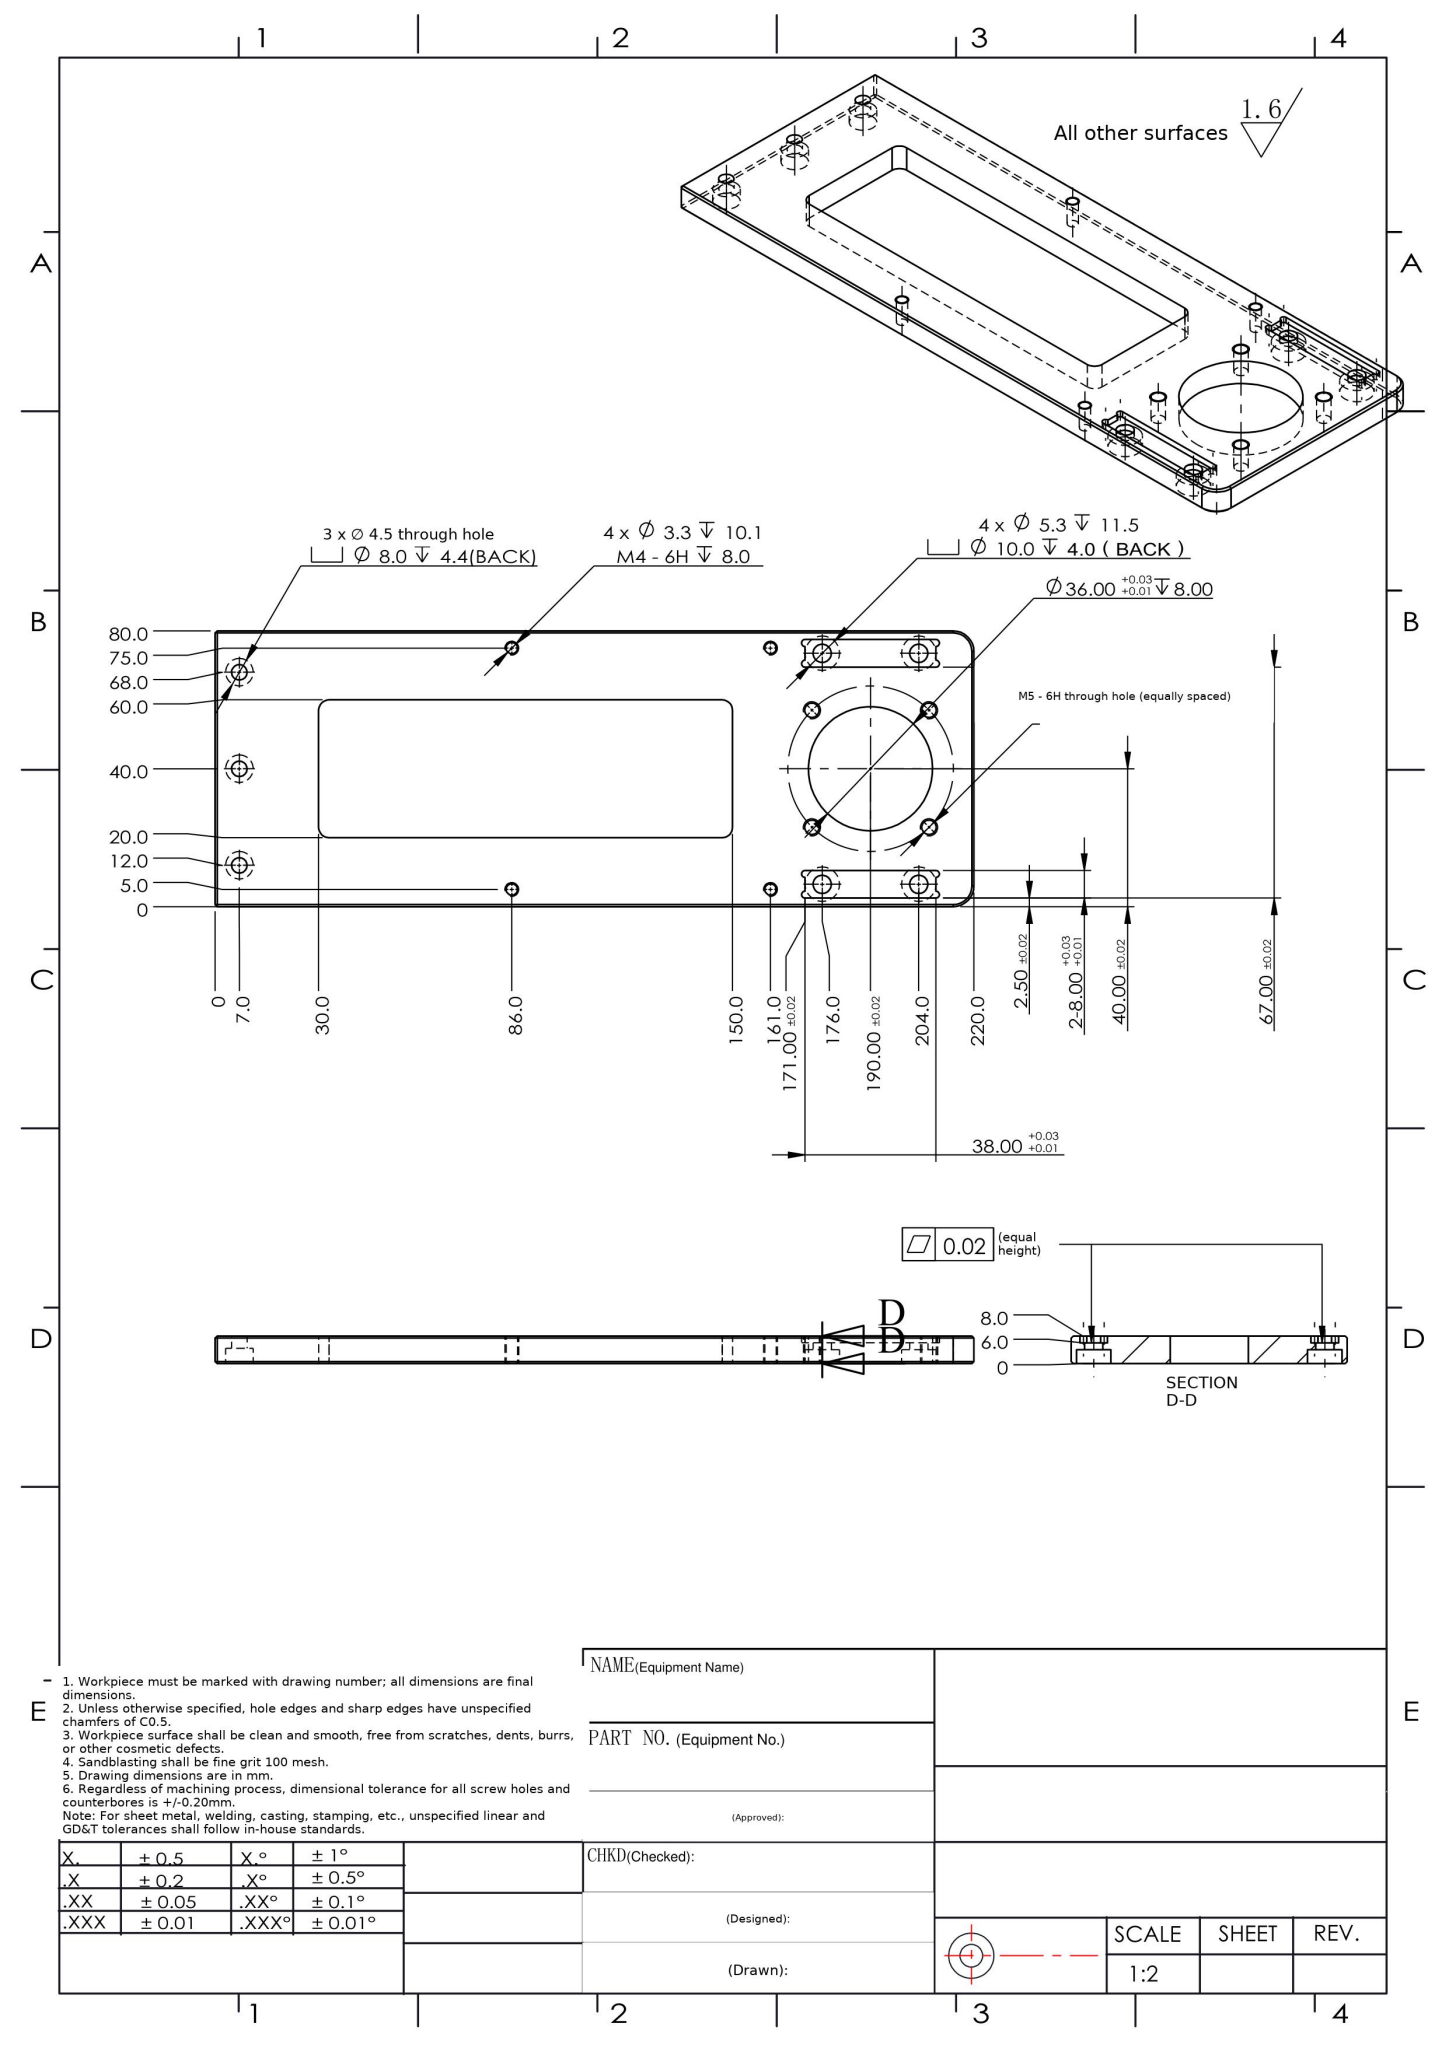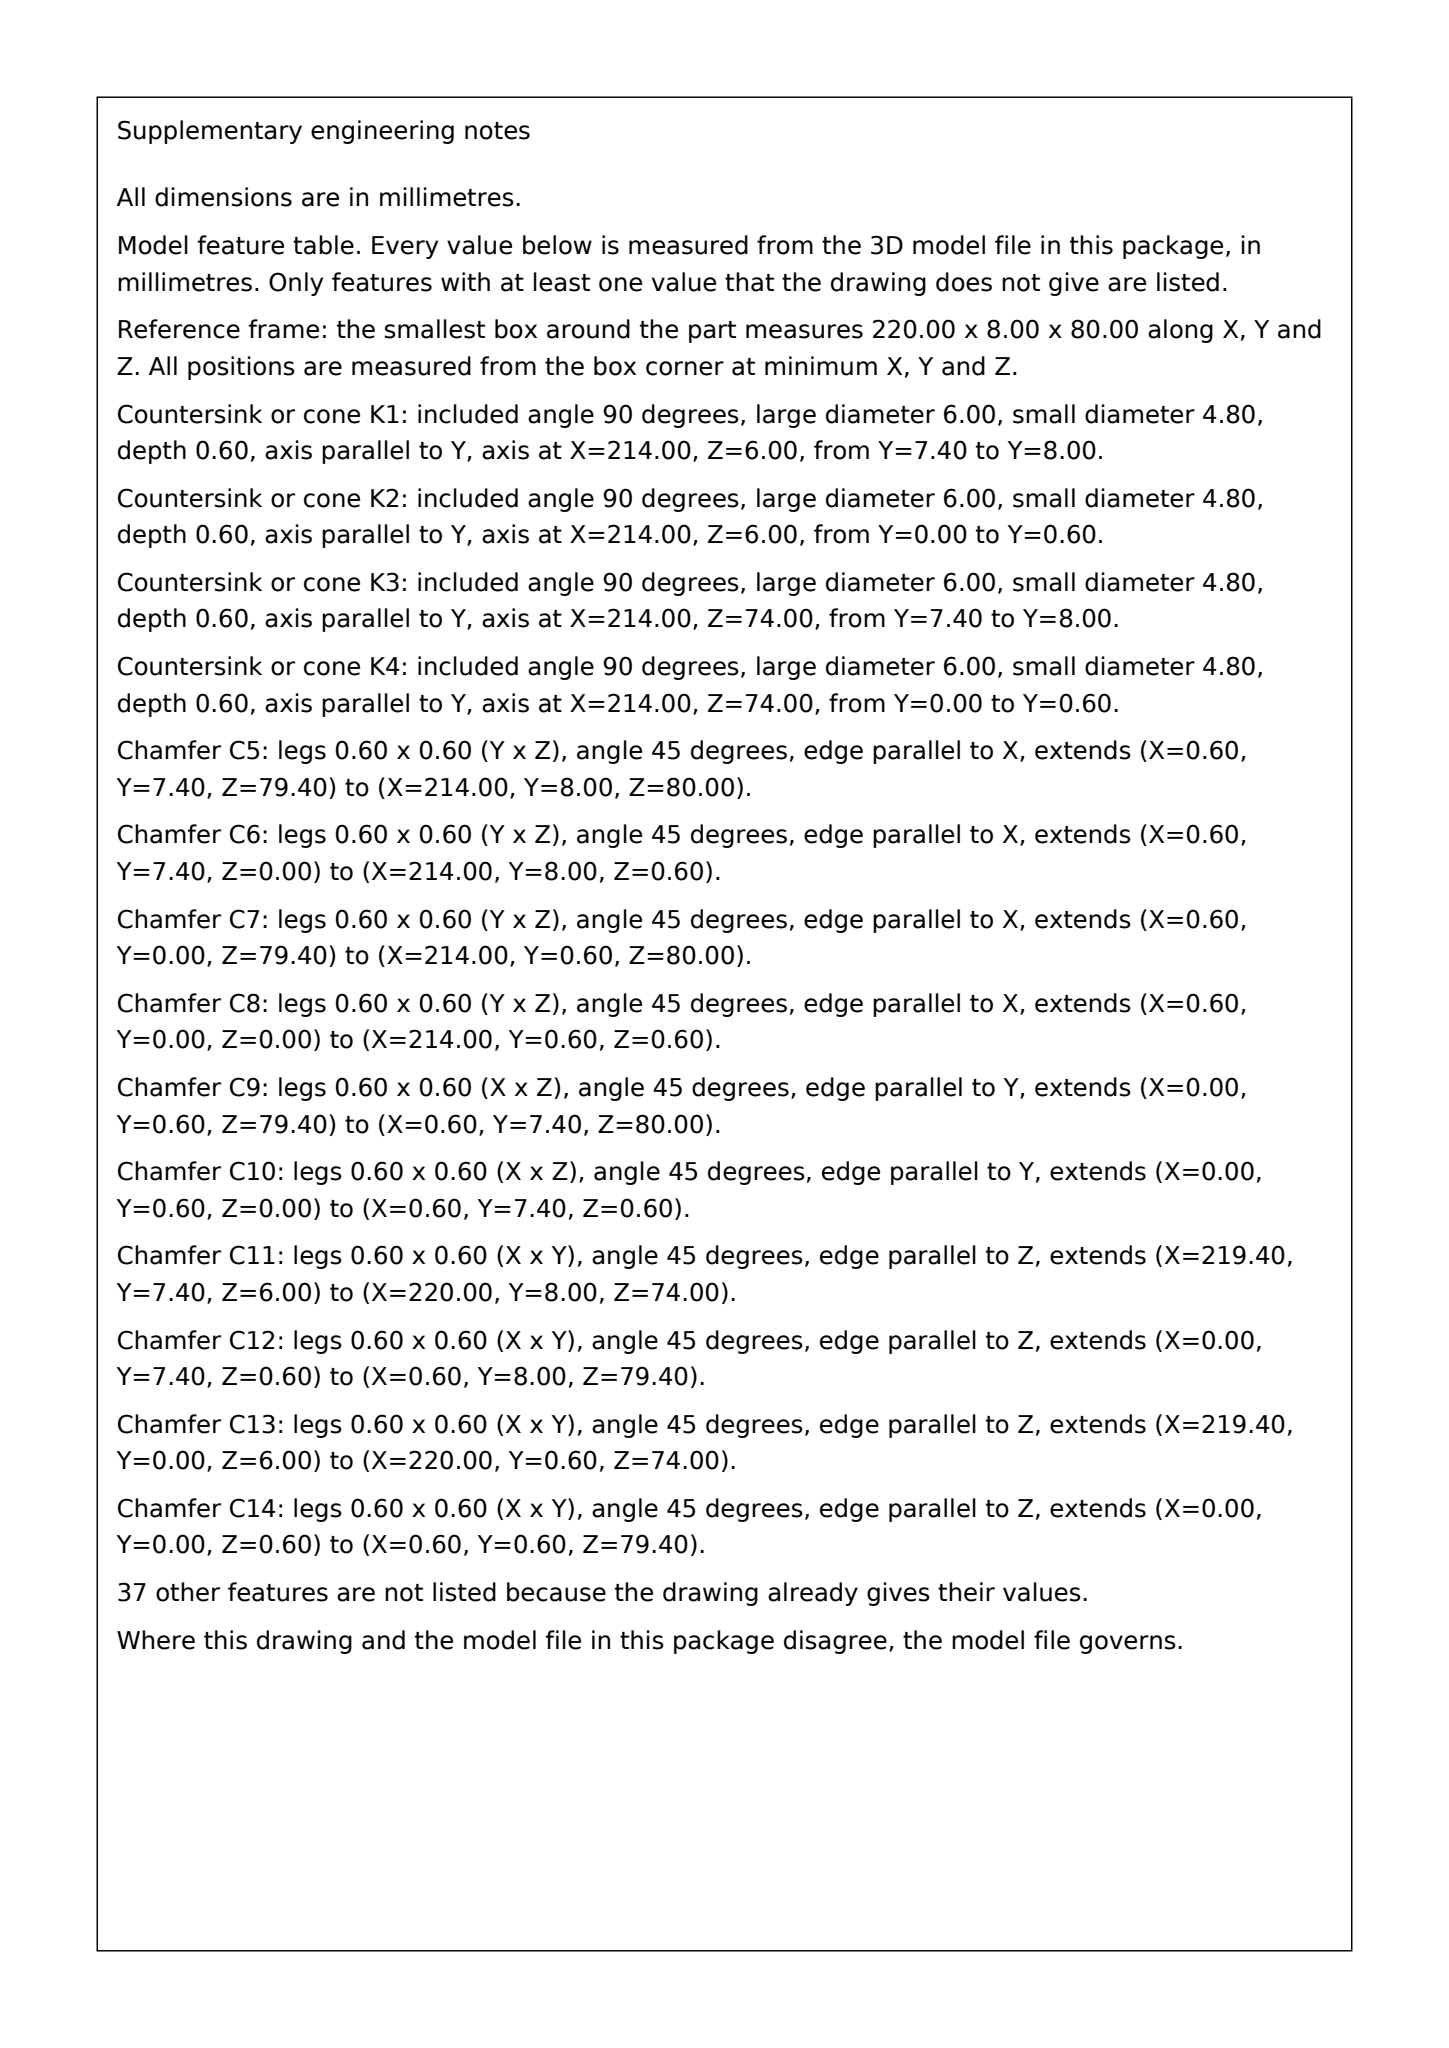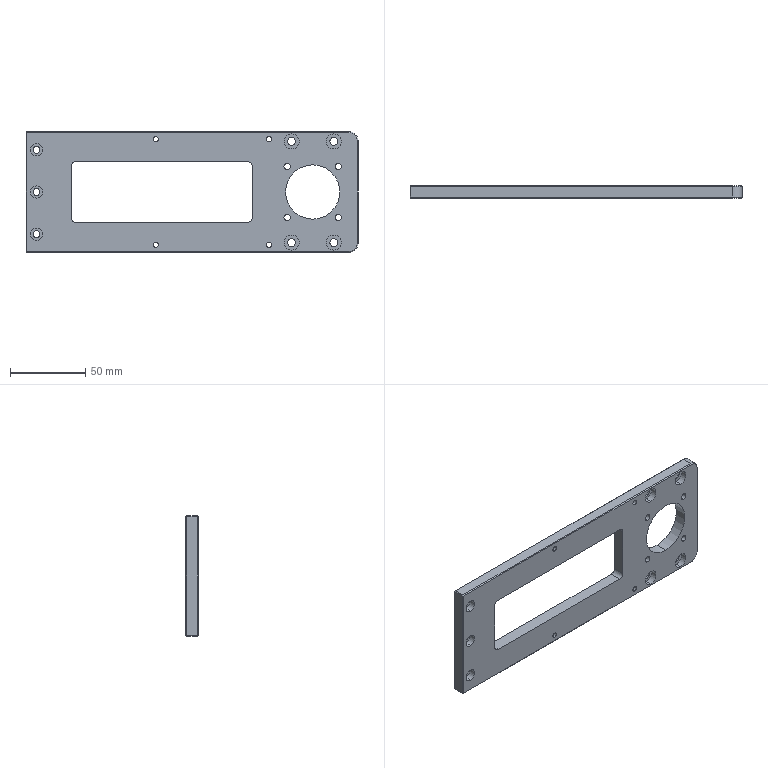Part | SolidWorks | mm | 1 solid | 105 faces | box 220 x 8 x 80 mm | volume 89752 mm3 | cylinder 60 | plane 41 | cone 4 | commonest cylinder face diameters 10 x8 5.3 x8 4.2 x8 3.3 x8 2 x8 8 x6 4.5 x6 6 x4